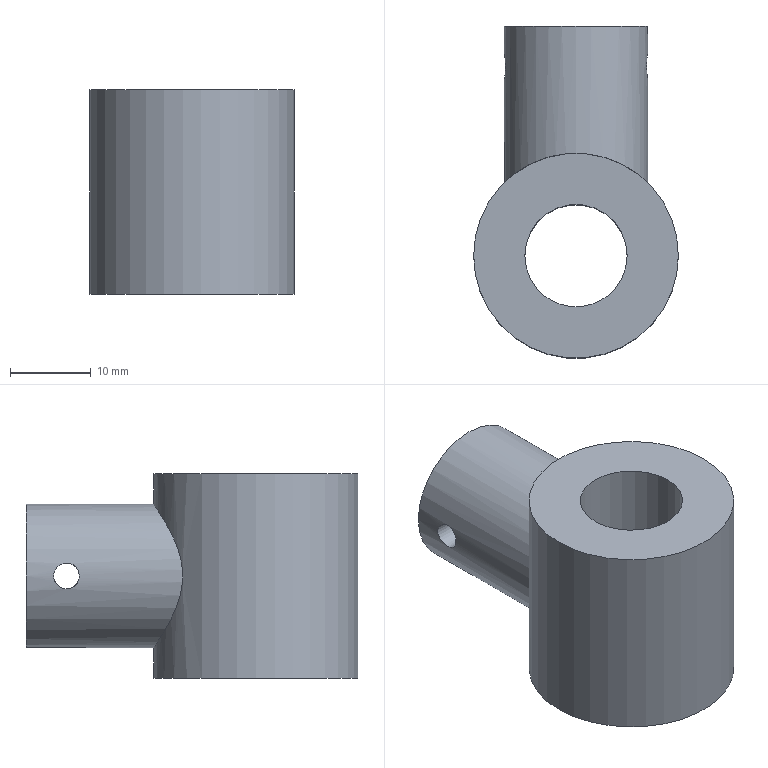Component | NX | SHAFT_SEAT | 1 solid | 7 faces | volume 13641 mm3 | cylinder 4 | plane 3 | commonest cylinder face diameters 25.4 x1 17.78 x1 3.2 x1 12.7 x1